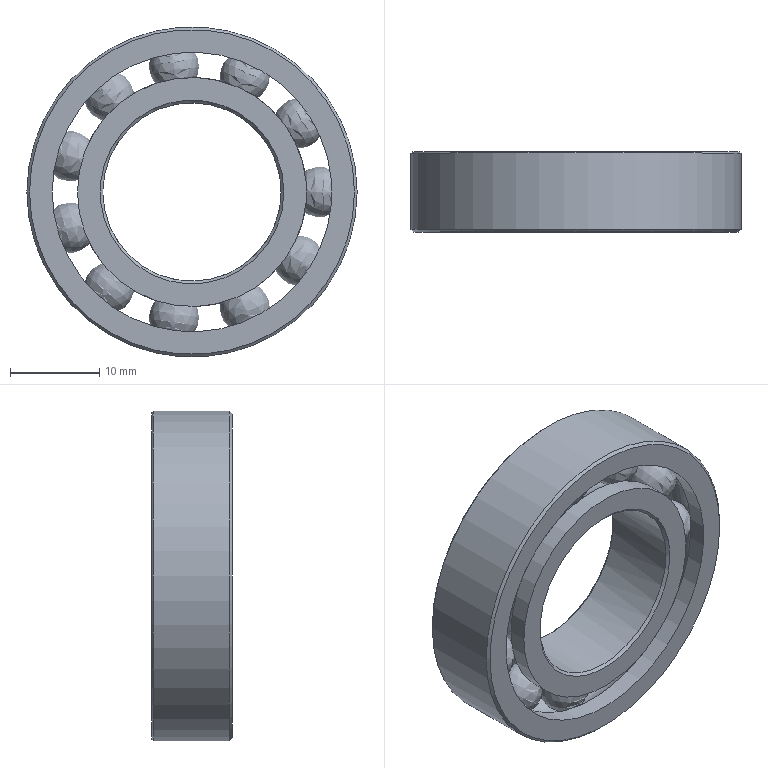Component | NX | GB-T292_C-1994_71904_C | 13 solids | 27 faces | volume 4662 mm3 | sphere 11 | cylinder 5 | cone 5 | plane 4 | torus 2 | commonest cylinder face diameters 25.667 x2 20 x1 37 x1 31.333 x1